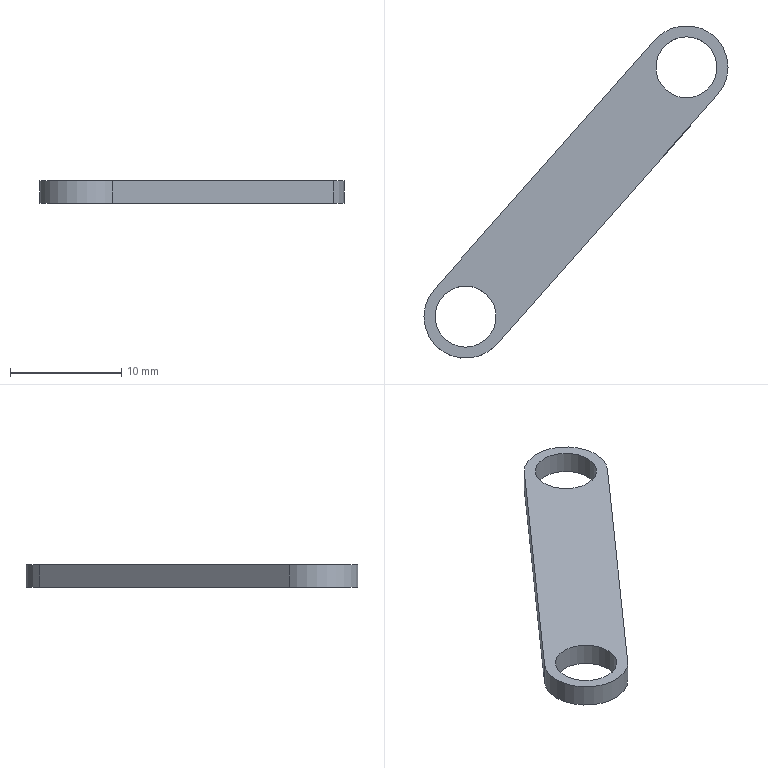Component | NX | CRANK_ROCKER_4 | 1 solid | 8 faces | box 27.39 x 29.96 x 2 mm | volume 443 mm3 | cylinder 4 | plane 4 | commonest cylinder face diameters 7.5 x2 5.5 x2
STEP:
#1=CARTESIAN_POINT('',(0.,0.,0.));
#2=DIRECTION('',(0.,0.,1.));
#3=DIRECTION('',(1.,0.,0.));
#4=AXIS2_PLACEMENT_3D('',#1,#2,#3);
#5=CARTESIAN_POINT('',(-7.307,4.198,-8.49));
#6=VERTEX_POINT('',#5);
#7=CARTESIAN_POINT('',(-12.921,9.171,-8.49));
#8=VERTEX_POINT('',#7);
#9=CARTESIAN_POINT('',(-10.114,6.685,-8.49));
#10=DIRECTION('',(0.,0.,1.));
#11=DIRECTION('',(-0.663,-0.7486,0.));
#12=AXIS2_PLACEMENT_3D('',#9,#10,#11);
#13=CIRCLE('',#12,3.75);
#14=CARTESIAN_POINT('',(-10.114,6.685,-6.49));
#15=DIRECTION('',(0.,0.,-1.));
#16=DIRECTION('',(0.663,0.7486,0.));
#17=AXIS2_PLACEMENT_3D('',#14,#15,#16);
#18=CYLINDRICAL_SURFACE('',#17,3.75);
#19=CARTESIAN_POINT('',(9.425,2.));
#20=DIRECTION('',(-1.,0.));
#21=VECTOR('',#20,1.);
#22=LINE('',#19,#21);
#23=(GEOMETRIC_REPRESENTATION_CONTEXT(2)PARAMETRIC_REPRESENTATION_CONTEXT()REPRESENTATION_CONTEXT('',''));
#24=DEFINITIONAL_REPRESENTATION('',(#22),#23);
#25=PCURVE('',#18,#24);
#26=CARTESIAN_POINT('',(-10.114,6.685,-8.49));
#27=DIRECTION('',(0.,0.,1.));
#28=DIRECTION('',(-0.663,-0.7486,0.));
#29=AXIS2_PLACEMENT_3D('',#26,#27,#28);
#30=PLANE('',#29);
#31=CARTESIAN_POINT('',(0.,0.));
#32=DIRECTION('',(1.,0.));
#33=AXIS2_PLACEMENT_2D('',#31,#32);
#34=CIRCLE('',#33,3.75);
#35=(GEOMETRIC_REPRESENTATION_CONTEXT(2)PARAMETRIC_REPRESENTATION_CONTEXT()REPRESENTATION_CONTEXT('',''));
#36=DEFINITIONAL_REPRESENTATION('',(#34),#35);
#37=PCURVE('',#30,#36);
#38=SURFACE_CURVE('',#13,(#25,#37),.PCURVE_S1.);
#39=EDGE_CURVE('',#6,#8,#38,.T.);
#40=ORIENTED_EDGE('',*,*,#39,.T.);
#41=CARTESIAN_POINT('',(-12.921,9.171,-6.49));
#42=VERTEX_POINT('',#41);
#43=CARTESIAN_POINT('',(-12.921,9.171,-6.49));
#44=DIRECTION('',(0.,0.,-1.));
#45=VECTOR('',#44,1.);
#46=LINE('',#43,#45);
#47=CARTESIAN_POINT('',(4.712,0.));
#48=DIRECTION('',(0.,1.));
#49=VECTOR('',#48,1.);
#50=LINE('',#47,#49);
#51=(GEOMETRIC_REPRESENTATION_CONTEXT(2)PARAMETRIC_REPRESENTATION_CONTEXT()REPRESENTATION_CONTEXT('',''));
#52=DEFINITIONAL_REPRESENTATION('',(#50),#51);
#53=PCURVE('',#18,#52);
#54=CARTESIAN_POINT('',(-12.921,9.171,-6.49));
#55=DIRECTION('',(0.7486,-0.663,0.));
#56=DIRECTION('',(0.663,0.7486,0.));
#57=AXIS2_PLACEMENT_3D('',#54,#55,#56);
#58=PLANE('',#57);
#59=CARTESIAN_POINT('',(0.,0.));
#60=DIRECTION('',(0.,-1.));
#61=VECTOR('',#60,1.);
#62=LINE('',#59,#61);
#63=(GEOMETRIC_REPRESENTATION_CONTEXT(2)PARAMETRIC_REPRESENTATION_CONTEXT()REPRESENTATION_CONTEXT('',''));
#64=DEFINITIONAL_REPRESENTATION('',(#62),#63);
#65=PCURVE('',#58,#64);
#66=SURFACE_CURVE('',#46,(#53,#65),.PCURVE_S1.);
#67=EDGE_CURVE('',#42,#8,#66,.T.);
#68=ORIENTED_EDGE('',*,*,#67,.F.);
#69=CARTESIAN_POINT('',(-7.307,4.198,-6.49));
#70=VERTEX_POINT('',#69);
#71=CARTESIAN_POINT('',(-10.114,6.685,-6.49));
#72=DIRECTION('',(0.,0.,1.));
#73=DIRECTION('',(-0.663,-0.7486,0.));
#74=AXIS2_PLACEMENT_3D('',#71,#72,#73);
#75=CIRCLE('',#74,3.75);
#76=CARTESIAN_POINT('',(9.425,0.));
#77=DIRECTION('',(-1.,0.));
#78=VECTOR('',#77,1.);
#79=LINE('',#76,#78);
#80=(GEOMETRIC_REPRESENTATION_CONTEXT(2)PARAMETRIC_REPRESENTATION_CONTEXT()REPRESENTATION_CONTEXT('',''));
#81=DEFINITIONAL_REPRESENTATION('',(#79),#80);
#82=PCURVE('',#18,#81);
#83=CARTESIAN_POINT('',(-10.114,6.685,-6.49));
#84=DIRECTION('',(0.,0.,1.));
#85=DIRECTION('',(-0.663,-0.7486,0.));
#86=AXIS2_PLACEMENT_3D('',#83,#84,#85);
#87=PLANE('',#86);
#88=CARTESIAN_POINT('',(0.,0.));
#89=DIRECTION('',(1.,0.));
#90=AXIS2_PLACEMENT_2D('',#88,#89);
#91=CIRCLE('',#90,3.75);
#92=(GEOMETRIC_REPRESENTATION_CONTEXT(2)PARAMETRIC_REPRESENTATION_CONTEXT()REPRESENTATION_CONTEXT('',''));
#93=DEFINITIONAL_REPRESENTATION('',(#91),#92);
#94=PCURVE('',#87,#93);
#95=SURFACE_CURVE('',#75,(#82,#94),.PCURVE_S1.);
#96=EDGE_CURVE('',#70,#42,#95,.T.);
#97=ORIENTED_EDGE('',*,*,#96,.F.);
#98=CARTESIAN_POINT('',(-7.307,4.198,-6.49));
#99=DIRECTION('',(0.,0.,-1.));
#100=VECTOR('',#99,1.);
#101=LINE('',#98,#100);
#102=CARTESIAN_POINT('',(7.854,0.));
#103=DIRECTION('',(0.,1.));
#104=VECTOR('',#103,1.);
#105=LINE('',#102,#104);
#106=(GEOMETRIC_REPRESENTATION_CONTEXT(2)PARAMETRIC_REPRESENTATION_CONTEXT()REPRESENTATION_CONTEXT('',''));
#107=DEFINITIONAL_REPRESENTATION('',(#105),#106);
#108=PCURVE('',#18,#107);
#109=CARTESIAN_POINT('',(-27.196,-18.261,-6.49));
#110=DIRECTION('',(-0.7486,0.663,0.));
#111=DIRECTION('',(-0.663,-0.7486,0.));
#112=AXIS2_PLACEMENT_3D('',#109,#110,#111);
#113=PLANE('',#112);
#114=CARTESIAN_POINT('',(-30.,0.));
#115=DIRECTION('',(0.,-1.));
#116=VECTOR('',#115,1.);
#117=LINE('',#114,#116);
#118=(GEOMETRIC_REPRESENTATION_CONTEXT(2)PARAMETRIC_REPRESENTATION_CONTEXT()REPRESENTATION_CONTEXT('',''));
#119=DEFINITIONAL_REPRESENTATION('',(#117),#118);
#120=PCURVE('',#113,#119);
#121=SURFACE_CURVE('',#101,(#108,#120),.PCURVE_S1.);
#122=EDGE_CURVE('',#70,#6,#121,.T.);
#123=ORIENTED_EDGE('',*,*,#122,.T.);
#124=EDGE_LOOP('',(#40,#68,#97,#123));
#125=FACE_BOUND('',#124,.T.);
#126=ADVANCED_FACE('',(#125),#18,.T.);
#127=CARTESIAN_POINT('',(-32.811,-13.288,-8.49));
#128=VERTEX_POINT('',#127);
#129=CARTESIAN_POINT('',(-12.921,9.171,-8.49));
#130=DIRECTION('',(-0.663,-0.7486,0.));
#131=VECTOR('',#130,1.);
#132=LINE('',#129,#131);
#133=CARTESIAN_POINT('',(0.,-2.));
#134=DIRECTION('',(-1.,0.));
#135=VECTOR('',#134,1.);
#136=LINE('',#133,#135);
#137=(GEOMETRIC_REPRESENTATION_CONTEXT(2)PARAMETRIC_REPRESENTATION_CONTEXT()REPRESENTATION_CONTEXT('',''));
#138=DEFINITIONAL_REPRESENTATION('',(#136),#137);
#139=PCURVE('',#58,#138);
#140=CARTESIAN_POINT('',(-0.,-3.75));
#141=DIRECTION('',(1.,0.));
#142=VECTOR('',#141,1.);
#143=LINE('',#140,#142);
#144=(GEOMETRIC_REPRESENTATION_CONTEXT(2)PARAMETRIC_REPRESENTATION_CONTEXT()REPRESENTATION_CONTEXT('',''));
#145=DEFINITIONAL_REPRESENTATION('',(#143),#144);
#146=PCURVE('',#30,#145);
#147=SURFACE_CURVE('',#132,(#139,#146),.PCURVE_S1.);
#148=EDGE_CURVE('',#8,#128,#147,.T.);
#149=ORIENTED_EDGE('',*,*,#148,.T.);
#150=CARTESIAN_POINT('',(-32.811,-13.288,-6.49));
#151=VERTEX_POINT('',#150);
#152=CARTESIAN_POINT('',(-32.811,-13.288,-6.49));
#153=DIRECTION('',(0.,0.,-1.));
#154=VECTOR('',#153,1.);
#155=LINE('',#152,#154);
#156=CARTESIAN_POINT('',(-30.,0.));
#157=DIRECTION('',(0.,-1.));
#158=VECTOR('',#157,1.);
#159=LINE('',#156,#158);
#160=(GEOMETRIC_REPRESENTATION_CONTEXT(2)PARAMETRIC_REPRESENTATION_CONTEXT()REPRESENTATION_CONTEXT('',''));
#161=DEFINITIONAL_REPRESENTATION('',(#159),#160);
#162=PCURVE('',#58,#161);
#163=CARTESIAN_POINT('',(-30.003,-15.774,-6.49));
#164=DIRECTION('',(0.,0.,-1.));
#165=DIRECTION('',(0.663,0.7486,0.));
#166=AXIS2_PLACEMENT_3D('',#163,#164,#165);
#167=CYLINDRICAL_SURFACE('',#166,3.75);
#168=CARTESIAN_POINT('',(4.712,0.));
#169=DIRECTION('',(0.,1.));
#170=VECTOR('',#169,1.);
#171=LINE('',#168,#170);
#172=(GEOMETRIC_REPRESENTATION_CONTEXT(2)PARAMETRIC_REPRESENTATION_CONTEXT()REPRESENTATION_CONTEXT('',''));
#173=DEFINITIONAL_REPRESENTATION('',(#171),#172);
#174=PCURVE('',#167,#173);
#175=SURFACE_CURVE('',#155,(#162,#174),.PCURVE_S1.);
#176=EDGE_CURVE('',#151,#128,#175,.T.);
#177=ORIENTED_EDGE('',*,*,#176,.F.);
#178=CARTESIAN_POINT('',(-12.921,9.171,-6.49));
#179=DIRECTION('',(-0.663,-0.7486,0.));
#180=VECTOR('',#179,1.);
#181=LINE('',#178,#180);
#182=CARTESIAN_POINT('',(0.,0.));
#183=DIRECTION('',(-1.,0.));
#184=VECTOR('',#183,1.);
#185=LINE('',#182,#184);
#186=(GEOMETRIC_REPRESENTATION_CONTEXT(2)PARAMETRIC_REPRESENTATION_CONTEXT()REPRESENTATION_CONTEXT('',''));
#187=DEFINITIONAL_REPRESENTATION('',(#185),#186);
#188=PCURVE('',#58,#187);
#189=CARTESIAN_POINT('',(-0.,-3.75));
#190=DIRECTION('',(1.,0.));
#191=VECTOR('',#190,1.);
#192=LINE('',#189,#191);
#193=(GEOMETRIC_REPRESENTATION_CONTEXT(2)PARAMETRIC_REPRESENTATION_CONTEXT()REPRESENTATION_CONTEXT('',''));
#194=DEFINITIONAL_REPRESENTATION('',(#192),#193);
#195=PCURVE('',#87,#194);
#196=SURFACE_CURVE('',#181,(#188,#195),.PCURVE_S1.);
#197=EDGE_CURVE('',#42,#151,#196,.T.);
#198=ORIENTED_EDGE('',*,*,#197,.F.);
#199=ORIENTED_EDGE('',*,*,#67,.T.);
#200=EDGE_LOOP('',(#149,#177,#198,#199));
#201=FACE_BOUND('',#200,.T.);
#202=ADVANCED_FACE('',(#201),#58,.F.);
#203=CARTESIAN_POINT('',(-27.196,-18.261,-8.49));
#204=VERTEX_POINT('',#203);
#205=CARTESIAN_POINT('',(-30.003,-15.774,-8.49));
#206=DIRECTION('',(0.,0.,1.));
#207=DIRECTION('',(-0.663,-0.7486,0.));
#208=AXIS2_PLACEMENT_3D('',#205,#206,#207);
#209=CIRCLE('',#208,3.75);
#210=CARTESIAN_POINT('',(9.425,2.));
#211=DIRECTION('',(-1.,0.));
#212=VECTOR('',#211,1.);
#213=LINE('',#210,#212);
#214=(GEOMETRIC_REPRESENTATION_CONTEXT(2)PARAMETRIC_REPRESENTATION_CONTEXT()REPRESENTATION_CONTEXT('',''));
#215=DEFINITIONAL_REPRESENTATION('',(#213),#214);
#216=PCURVE('',#167,#215);
#217=CARTESIAN_POINT('',(30.,0.));
#218=DIRECTION('',(1.,0.));
#219=AXIS2_PLACEMENT_2D('',#217,#218);
#220=CIRCLE('',#219,3.75);
#221=(GEOMETRIC_REPRESENTATION_CONTEXT(2)PARAMETRIC_REPRESENTATION_CONTEXT()REPRESENTATION_CONTEXT('',''));
#222=DEFINITIONAL_REPRESENTATION('',(#220),#221);
#223=PCURVE('',#30,#222);
#224=SURFACE_CURVE('',#209,(#216,#223),.PCURVE_S1.);
#225=EDGE_CURVE('',#128,#204,#224,.T.);
#226=ORIENTED_EDGE('',*,*,#225,.T.);
#227=CARTESIAN_POINT('',(-27.196,-18.261,-6.49));
#228=VERTEX_POINT('',#227);
#229=CARTESIAN_POINT('',(-27.196,-18.261,-6.49));
#230=DIRECTION('',(0.,0.,-1.));
#231=VECTOR('',#230,1.);
#232=LINE('',#229,#231);
#233=CARTESIAN_POINT('',(1.571,0.));
#234=DIRECTION('',(0.,1.));
#235=VECTOR('',#234,1.);
#236=LINE('',#233,#235);
#237=(GEOMETRIC_REPRESENTATION_CONTEXT(2)PARAMETRIC_REPRESENTATION_CONTEXT()REPRESENTATION_CONTEXT('',''));
#238=DEFINITIONAL_REPRESENTATION('',(#236),#237);
#239=PCURVE('',#167,#238);
#240=CARTESIAN_POINT('',(0.,0.));
#241=DIRECTION('',(0.,-1.));
#242=VECTOR('',#241,1.);
#243=LINE('',#240,#242);
#244=(GEOMETRIC_REPRESENTATION_CONTEXT(2)PARAMETRIC_REPRESENTATION_CONTEXT()REPRESENTATION_CONTEXT('',''));
#245=DEFINITIONAL_REPRESENTATION('',(#243),#244);
#246=PCURVE('',#113,#245);
#247=SURFACE_CURVE('',#232,(#239,#246),.PCURVE_S1.);
#248=EDGE_CURVE('',#228,#204,#247,.T.);
#249=ORIENTED_EDGE('',*,*,#248,.F.);
#250=CARTESIAN_POINT('',(-30.003,-15.774,-6.49));
#251=DIRECTION('',(0.,0.,1.));
#252=DIRECTION('',(-0.663,-0.7486,0.));
#253=AXIS2_PLACEMENT_3D('',#250,#251,#252);
#254=CIRCLE('',#253,3.75);
#255=CARTESIAN_POINT('',(9.425,0.));
#256=DIRECTION('',(-1.,0.));
#257=VECTOR('',#256,1.);
#258=LINE('',#255,#257);
#259=(GEOMETRIC_REPRESENTATION_CONTEXT(2)PARAMETRIC_REPRESENTATION_CONTEXT()REPRESENTATION_CONTEXT('',''));
#260=DEFINITIONAL_REPRESENTATION('',(#258),#259);
#261=PCURVE('',#167,#260);
#262=CARTESIAN_POINT('',(30.,0.));
#263=DIRECTION('',(1.,0.));
#264=AXIS2_PLACEMENT_2D('',#262,#263);
#265=CIRCLE('',#264,3.75);
#266=(GEOMETRIC_REPRESENTATION_CONTEXT(2)PARAMETRIC_REPRESENTATION_CONTEXT()REPRESENTATION_CONTEXT('',''));
#267=DEFINITIONAL_REPRESENTATION('',(#265),#266);
#268=PCURVE('',#87,#267);
#269=SURFACE_CURVE('',#254,(#261,#268),.PCURVE_S1.);
#270=EDGE_CURVE('',#151,#228,#269,.T.);
#271=ORIENTED_EDGE('',*,*,#270,.F.);
#272=ORIENTED_EDGE('',*,*,#176,.T.);
#273=EDGE_LOOP('',(#226,#249,#271,#272));
#274=FACE_BOUND('',#273,.T.);
#275=ADVANCED_FACE('',(#274),#167,.T.);
#276=CARTESIAN_POINT('',(-11.937,4.626,-6.49));
#277=VERTEX_POINT('',#276);
#278=CARTESIAN_POINT('',(-10.114,6.685,-6.49));
#279=DIRECTION('',(0.,0.,1.));
#280=DIRECTION('',(-0.663,-0.7486,0.));
#281=AXIS2_PLACEMENT_3D('',#278,#279,#280);
#282=CIRCLE('',#281,2.75);
#283=CARTESIAN_POINT('',(-10.114,6.685,-6.49));
#284=DIRECTION('',(0.,0.,-1.));
#285=DIRECTION('',(0.663,0.7486,0.));
#286=AXIS2_PLACEMENT_3D('',#283,#284,#285);
#287=CYLINDRICAL_SURFACE('',#286,2.75);
#288=CARTESIAN_POINT('',(9.425,0.));
#289=DIRECTION('',(-1.,0.));
#290=VECTOR('',#289,1.);
#291=LINE('',#288,#290);
#292=(GEOMETRIC_REPRESENTATION_CONTEXT(2)PARAMETRIC_REPRESENTATION_CONTEXT()REPRESENTATION_CONTEXT('',''));
#293=DEFINITIONAL_REPRESENTATION('',(#291),#292);
#294=PCURVE('',#287,#293);
#295=CARTESIAN_POINT('',(0.,0.));
#296=DIRECTION('',(1.,0.));
#297=AXIS2_PLACEMENT_2D('',#295,#296);
#298=CIRCLE('',#297,2.75);
#299=(GEOMETRIC_REPRESENTATION_CONTEXT(2)PARAMETRIC_REPRESENTATION_CONTEXT()REPRESENTATION_CONTEXT('',''));
#300=DEFINITIONAL_REPRESENTATION('',(#298),#299);
#301=PCURVE('',#87,#300);
#302=SURFACE_CURVE('',#282,(#294,#301),.PCURVE_S1.);
#303=EDGE_CURVE('',#277,#277,#302,.T.);
#304=ORIENTED_EDGE('',*,*,#303,.F.);
#305=CARTESIAN_POINT('',(-11.937,4.626,-8.49));
#306=VERTEX_POINT('',#305);
#307=CARTESIAN_POINT('',(-11.937,4.626,-6.49));
#308=CARTESIAN_POINT('',(-11.937,4.626,-8.49));
#309=B_SPLINE_CURVE_WITH_KNOTS('',1,(#307,#308),.UNSPECIFIED.,.F.,.F.,(2,2),(0.,2.),.PIECEWISE_BEZIER_KNOTS.);
#310=CARTESIAN_POINT('',(9.425,0.));
#311=DIRECTION('',(0.,1.));
#312=VECTOR('',#311,1.);
#313=LINE('',#310,#312);
#314=(GEOMETRIC_REPRESENTATION_CONTEXT(2)PARAMETRIC_REPRESENTATION_CONTEXT()REPRESENTATION_CONTEXT('',''));
#315=DEFINITIONAL_REPRESENTATION('',(#313),#314);
#316=PCURVE('',#287,#315);
#317=CARTESIAN_POINT('',(3.142,0.));
#318=DIRECTION('',(0.,1.));
#319=VECTOR('',#318,1.);
#320=LINE('',#317,#319);
#321=(GEOMETRIC_REPRESENTATION_CONTEXT(2)PARAMETRIC_REPRESENTATION_CONTEXT()REPRESENTATION_CONTEXT('',''));
#322=DEFINITIONAL_REPRESENTATION('',(#320),#321);
#323=PCURVE('',#287,#322);
#324=SEAM_CURVE('',#309,(#316,#323),.PCURVE_S1.);
#325=EDGE_CURVE('',#277,#306,#324,.T.);
#326=ORIENTED_EDGE('',*,*,#325,.T.);
#327=CARTESIAN_POINT('',(-10.114,6.685,-8.49));
#328=DIRECTION('',(0.,0.,1.));
#329=DIRECTION('',(-0.663,-0.7486,0.));
#330=AXIS2_PLACEMENT_3D('',#327,#328,#329);
#331=CIRCLE('',#330,2.75);
#332=CARTESIAN_POINT('',(9.425,2.));
#333=DIRECTION('',(-1.,0.));
#334=VECTOR('',#333,1.);
#335=LINE('',#332,#334);
#336=(GEOMETRIC_REPRESENTATION_CONTEXT(2)PARAMETRIC_REPRESENTATION_CONTEXT()REPRESENTATION_CONTEXT('',''));
#337=DEFINITIONAL_REPRESENTATION('',(#335),#336);
#338=PCURVE('',#287,#337);
#339=CARTESIAN_POINT('',(0.,0.));
#340=DIRECTION('',(1.,0.));
#341=AXIS2_PLACEMENT_2D('',#339,#340);
#342=CIRCLE('',#341,2.75);
#343=(GEOMETRIC_REPRESENTATION_CONTEXT(2)PARAMETRIC_REPRESENTATION_CONTEXT()REPRESENTATION_CONTEXT('',''));
#344=DEFINITIONAL_REPRESENTATION('',(#342),#343);
#345=PCURVE('',#30,#344);
#346=SURFACE_CURVE('',#331,(#338,#345),.PCURVE_S1.);
#347=EDGE_CURVE('',#306,#306,#346,.T.);
#348=ORIENTED_EDGE('',*,*,#347,.T.);
#349=ORIENTED_EDGE('',*,*,#325,.F.);
#350=EDGE_LOOP('',(#304,#326,#348,#349));
#351=FACE_BOUND('',#350,.F.);
#352=ADVANCED_FACE('',(#351),#287,.F.);
#353=CARTESIAN_POINT('',(-27.196,-18.261,-8.49));
#354=DIRECTION('',(0.663,0.7486,0.));
#355=VECTOR('',#354,1.);
#356=LINE('',#353,#355);
#357=CARTESIAN_POINT('',(0.,-2.));
#358=DIRECTION('',(-1.,0.));
#359=VECTOR('',#358,1.);
#360=LINE('',#357,#359);
#361=(GEOMETRIC_REPRESENTATION_CONTEXT(2)PARAMETRIC_REPRESENTATION_CONTEXT()REPRESENTATION_CONTEXT('',''));
#362=DEFINITIONAL_REPRESENTATION('',(#360),#361);
#363=PCURVE('',#113,#362);
#364=CARTESIAN_POINT('',(30.,3.75));
#365=DIRECTION('',(-1.,0.));
#366=VECTOR('',#365,1.);
#367=LINE('',#364,#366);
#368=(GEOMETRIC_REPRESENTATION_CONTEXT(2)PARAMETRIC_REPRESENTATION_CONTEXT()REPRESENTATION_CONTEXT('',''));
#369=DEFINITIONAL_REPRESENTATION('',(#367),#368);
#370=PCURVE('',#30,#369);
#371=SURFACE_CURVE('',#356,(#363,#370),.PCURVE_S1.);
#372=EDGE_CURVE('',#204,#6,#371,.T.);
#373=ORIENTED_EDGE('',*,*,#372,.T.);
#374=ORIENTED_EDGE('',*,*,#122,.F.);
#375=CARTESIAN_POINT('',(-27.196,-18.261,-6.49));
#376=DIRECTION('',(0.663,0.7486,0.));
#377=VECTOR('',#376,1.);
#378=LINE('',#375,#377);
#379=CARTESIAN_POINT('',(0.,0.));
#380=DIRECTION('',(-1.,0.));
#381=VECTOR('',#380,1.);
#382=LINE('',#379,#381);
#383=(GEOMETRIC_REPRESENTATION_CONTEXT(2)PARAMETRIC_REPRESENTATION_CONTEXT()REPRESENTATION_CONTEXT('',''));
#384=DEFINITIONAL_REPRESENTATION('',(#382),#383);
#385=PCURVE('',#113,#384);
#386=CARTESIAN_POINT('',(30.,3.75));
#387=DIRECTION('',(-1.,0.));
#388=VECTOR('',#387,1.);
#389=LINE('',#386,#388);
#390=(GEOMETRIC_REPRESENTATION_CONTEXT(2)PARAMETRIC_REPRESENTATION_CONTEXT()REPRESENTATION_CONTEXT('',''));
#391=DEFINITIONAL_REPRESENTATION('',(#389),#390);
#392=PCURVE('',#87,#391);
#393=SURFACE_CURVE('',#378,(#385,#392),.PCURVE_S1.);
#394=EDGE_CURVE('',#228,#70,#393,.T.);
#395=ORIENTED_EDGE('',*,*,#394,.F.);
#396=ORIENTED_EDGE('',*,*,#248,.T.);
#397=EDGE_LOOP('',(#373,#374,#395,#396));
#398=FACE_BOUND('',#397,.T.);
#399=ADVANCED_FACE('',(#398),#113,.F.);
#400=CARTESIAN_POINT('',(-31.826,-17.833,-6.49));
#401=VERTEX_POINT('',#400);
#402=CARTESIAN_POINT('',(-30.003,-15.774,-6.49));
#403=DIRECTION('',(0.,0.,1.));
#404=DIRECTION('',(-0.663,-0.7486,0.));
#405=AXIS2_PLACEMENT_3D('',#402,#403,#404);
#406=CIRCLE('',#405,2.75);
#407=CARTESIAN_POINT('',(-30.003,-15.774,-6.49));
#408=DIRECTION('',(0.,0.,-1.));
#409=DIRECTION('',(0.663,0.7486,0.));
#410=AXIS2_PLACEMENT_3D('',#407,#408,#409);
#411=CYLINDRICAL_SURFACE('',#410,2.75);
#412=CARTESIAN_POINT('',(9.425,0.));
#413=DIRECTION('',(-1.,0.));
#414=VECTOR('',#413,1.);
#415=LINE('',#412,#414);
#416=(GEOMETRIC_REPRESENTATION_CONTEXT(2)PARAMETRIC_REPRESENTATION_CONTEXT()REPRESENTATION_CONTEXT('',''));
#417=DEFINITIONAL_REPRESENTATION('',(#415),#416);
#418=PCURVE('',#411,#417);
#419=CARTESIAN_POINT('',(30.,0.));
#420=DIRECTION('',(1.,0.));
#421=AXIS2_PLACEMENT_2D('',#419,#420);
#422=CIRCLE('',#421,2.75);
#423=(GEOMETRIC_REPRESENTATION_CONTEXT(2)PARAMETRIC_REPRESENTATION_CONTEXT()REPRESENTATION_CONTEXT('',''));
#424=DEFINITIONAL_REPRESENTATION('',(#422),#423);
#425=PCURVE('',#87,#424);
#426=SURFACE_CURVE('',#406,(#418,#425),.PCURVE_S1.);
#427=EDGE_CURVE('',#401,#401,#426,.T.);
#428=ORIENTED_EDGE('',*,*,#427,.F.);
#429=CARTESIAN_POINT('',(-31.826,-17.833,-8.49));
#430=VERTEX_POINT('',#429);
#431=CARTESIAN_POINT('',(-31.826,-17.833,-6.49));
#432=CARTESIAN_POINT('',(-31.826,-17.833,-8.49));
#433=B_SPLINE_CURVE_WITH_KNOTS('',1,(#431,#432),.UNSPECIFIED.,.F.,.F.,(2,2),(0.,2.),.PIECEWISE_BEZIER_KNOTS.);
#434=CARTESIAN_POINT('',(9.425,0.));
#435=DIRECTION('',(0.,1.));
#436=VECTOR('',#435,1.);
#437=LINE('',#434,#436);
#438=(GEOMETRIC_REPRESENTATION_CONTEXT(2)PARAMETRIC_REPRESENTATION_CONTEXT()REPRESENTATION_CONTEXT('',''));
#439=DEFINITIONAL_REPRESENTATION('',(#437),#438);
#440=PCURVE('',#411,#439);
#441=CARTESIAN_POINT('',(3.142,0.));
#442=DIRECTION('',(0.,1.));
#443=VECTOR('',#442,1.);
#444=LINE('',#441,#443);
#445=(GEOMETRIC_REPRESENTATION_CONTEXT(2)PARAMETRIC_REPRESENTATION_CONTEXT()REPRESENTATION_CONTEXT('',''));
#446=DEFINITIONAL_REPRESENTATION('',(#444),#445);
#447=PCURVE('',#411,#446);
#448=SEAM_CURVE('',#433,(#440,#447),.PCURVE_S1.);
#449=EDGE_CURVE('',#401,#430,#448,.T.);
#450=ORIENTED_EDGE('',*,*,#449,.T.);
#451=CARTESIAN_POINT('',(-30.003,-15.774,-8.49));
#452=DIRECTION('',(0.,0.,1.));
#453=DIRECTION('',(-0.663,-0.7486,0.));
#454=AXIS2_PLACEMENT_3D('',#451,#452,#453);
#455=CIRCLE('',#454,2.75);
#456=CARTESIAN_POINT('',(9.425,2.));
#457=DIRECTION('',(-1.,0.));
#458=VECTOR('',#457,1.);
#459=LINE('',#456,#458);
#460=(GEOMETRIC_REPRESENTATION_CONTEXT(2)PARAMETRIC_REPRESENTATION_CONTEXT()REPRESENTATION_CONTEXT('',''));
#461=DEFINITIONAL_REPRESENTATION('',(#459),#460);
#462=PCURVE('',#411,#461);
#463=CARTESIAN_POINT('',(30.,0.));
#464=DIRECTION('',(1.,0.));
#465=AXIS2_PLACEMENT_2D('',#463,#464);
#466=CIRCLE('',#465,2.75);
#467=(GEOMETRIC_REPRESENTATION_CONTEXT(2)PARAMETRIC_REPRESENTATION_CONTEXT()REPRESENTATION_CONTEXT('',''));
#468=DEFINITIONAL_REPRESENTATION('',(#466),#467);
#469=PCURVE('',#30,#468);
#470=SURFACE_CURVE('',#455,(#462,#469),.PCURVE_S1.);
#471=EDGE_CURVE('',#430,#430,#470,.T.);
#472=ORIENTED_EDGE('',*,*,#471,.T.);
#473=ORIENTED_EDGE('',*,*,#449,.F.);
#474=EDGE_LOOP('',(#428,#450,#472,#473));
#475=FACE_BOUND('',#474,.F.);
#476=ADVANCED_FACE('',(#475),#411,.F.);
#477=ORIENTED_EDGE('',*,*,#96,.T.);
#478=ORIENTED_EDGE('',*,*,#197,.T.);
#479=ORIENTED_EDGE('',*,*,#270,.T.);
#480=ORIENTED_EDGE('',*,*,#394,.T.);
#481=EDGE_LOOP('',(#477,#478,#479,#480));
#482=FACE_BOUND('',#481,.T.);
#483=ORIENTED_EDGE('',*,*,#303,.F.);
#484=EDGE_LOOP('',(#483));
#485=FACE_BOUND('',#484,.T.);
#486=ORIENTED_EDGE('',*,*,#427,.F.);
#487=EDGE_LOOP('',(#486));
#488=FACE_BOUND('',#487,.T.);
#489=ADVANCED_FACE('',(#482,#485,#488),#87,.T.);
#490=ORIENTED_EDGE('',*,*,#39,.F.);
#491=ORIENTED_EDGE('',*,*,#372,.F.);
#492=ORIENTED_EDGE('',*,*,#225,.F.);
#493=ORIENTED_EDGE('',*,*,#148,.F.);
#494=EDGE_LOOP('',(#490,#491,#492,#493));
#495=FACE_BOUND('',#494,.T.);
#496=ORIENTED_EDGE('',*,*,#347,.T.);
#497=EDGE_LOOP('',(#496));
#498=FACE_BOUND('',#497,.T.);
#499=ORIENTED_EDGE('',*,*,#471,.T.);
#500=EDGE_LOOP('',(#499));
#501=FACE_BOUND('',#500,.T.);
#502=ADVANCED_FACE('',(#495,#498,#501),#30,.F.);
#503=CLOSED_SHELL('',(#126,#202,#275,#352,#399,#476,#489,#502));
#504=MANIFOLD_SOLID_BREP('',#503);
#505=(LENGTH_UNIT()NAMED_UNIT(*)SI_UNIT(.MILLI.,.METRE.));
#506=UNCERTAINTY_MEASURE_WITH_UNIT(LENGTH_MEASURE(0.000002),#505,'','');
#507=(NAMED_UNIT(*)PLANE_ANGLE_UNIT()SI_UNIT($,.RADIAN.));
#508=(NAMED_UNIT(*)SI_UNIT($,.STERADIAN.)SOLID_ANGLE_UNIT());
#509=(GEOMETRIC_REPRESENTATION_CONTEXT(3)GLOBAL_UNCERTAINTY_ASSIGNED_CONTEXT((#506))GLOBAL_UNIT_ASSIGNED_CONTEXT((#505,#507,#508))REPRESENTATION_CONTEXT('',''));
#510=ADVANCED_BREP_SHAPE_REPRESENTATION('',(#4,#504),#509);